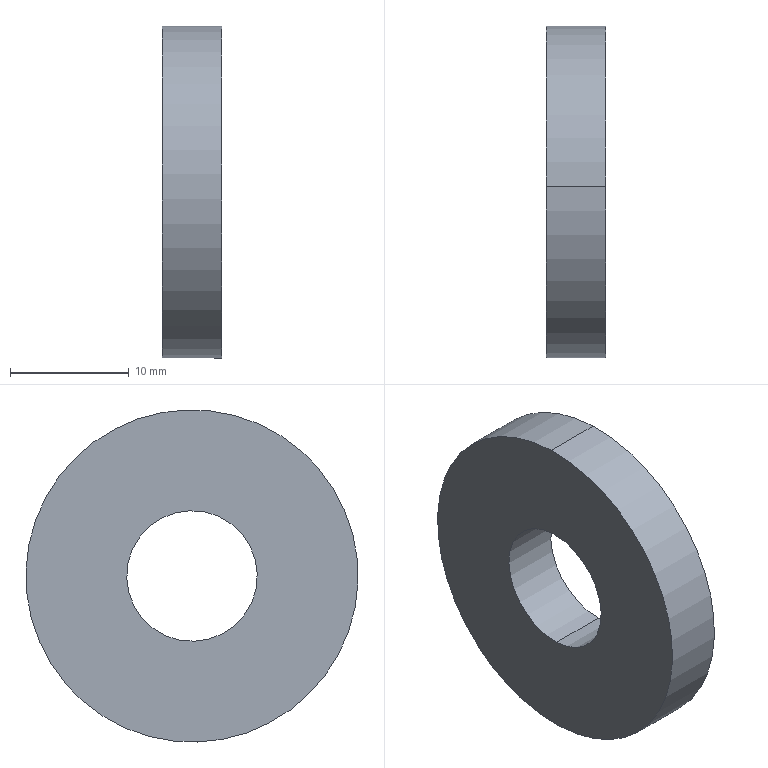Component | SolidWorks | Gasket-2 | 1 solid | 6 faces | box 5 x 28 x 28 mm | volume 2604 mm3 | cylinder 4 | plane 2 | commonest cylinder face diameters 11 x2 28 x2
build123d program:
from build123d import *

# Parameters (mm, degrees)
SKETCH1_R           = 14
SKETCH1_R_2         = 5.5
BOSS_EXTRUDE1_DEPTH = 5


with BuildPart() as part:
    # Sketch1 → Boss-Extrude1 (new body)
    with BuildSketch(Plane.XY):
        Circle(SKETCH1_R)
        Circle(SKETCH1_R_2, mode=Mode.SUBTRACT)
    extrude(amount=BOSS_EXTRUDE1_DEPTH)


solid = part.part

# Placed as in the assembly
solid = solid.moved(Location((-553.364, 0, 0), (0, 90, 0)))
STEP:
#1=CARTESIAN_POINT('',(-21.589,0.007104,0.2164));
#2=VERTEX_POINT('',#1);
#3=CARTESIAN_POINT('',(-21.589,-0.007104,-0.2164));
#4=VERTEX_POINT('',#3);
#5=CARTESIAN_POINT('',(-21.589,0.,0.));
#6=DIRECTION('',(1.,-0.,-0.));
#7=DIRECTION('',(0.,-0.03281,-0.9995));
#8=AXIS2_PLACEMENT_3D('',#5,#6,#7);
#9=CIRCLE('',#8,0.2165);
#10=EDGE_CURVE('',#2,#4,#9,.T.);
#11=ORIENTED_EDGE('',*,*,#10,.T.);
#12=CARTESIAN_POINT('',(-21.786,-0.007104,-0.2164));
#13=VERTEX_POINT('',#12);
#14=CARTESIAN_POINT('',(-21.589,-0.007104,-0.2164));
#15=DIRECTION('',(-1.,0.,0.));
#16=VECTOR('',#15,39.37);
#17=LINE('',#14,#16);
#18=EDGE_CURVE('',#4,#13,#17,.T.);
#19=ORIENTED_EDGE('',*,*,#18,.T.);
#20=CARTESIAN_POINT('',(-21.786,0.007104,0.2164));
#21=VERTEX_POINT('',#20);
#22=CARTESIAN_POINT('',(-21.786,0.,0.));
#23=DIRECTION('',(1.,-0.,-0.));
#24=DIRECTION('',(0.,-0.03281,-0.9995));
#25=AXIS2_PLACEMENT_3D('',#22,#23,#24);
#26=CIRCLE('',#25,0.2165);
#27=EDGE_CURVE('',#21,#13,#26,.T.);
#28=ORIENTED_EDGE('',*,*,#27,.F.);
#29=CARTESIAN_POINT('',(-21.589,0.007104,0.2164));
#30=DIRECTION('',(-1.,0.,0.));
#31=VECTOR('',#30,39.37);
#32=LINE('',#29,#31);
#33=EDGE_CURVE('',#2,#21,#32,.T.);
#34=ORIENTED_EDGE('',*,*,#33,.F.);
#35=EDGE_LOOP('',(#11,#19,#28,#34));
#36=FACE_OUTER_BOUND('',#35,.T.);
#37=CARTESIAN_POINT('',(-21.589,0.,0.));
#38=DIRECTION('',(-1.,0.,0.));
#39=DIRECTION('',(0.,0.03281,0.9995));
#40=AXIS2_PLACEMENT_3D('',#37,#38,#39);
#41=CYLINDRICAL_SURFACE('',#40,0.2165);
#42=ADVANCED_FACE('',(#36),#41,.F.);
#43=CARTESIAN_POINT('',(-21.589,-0.01808,-0.5509));
#44=VERTEX_POINT('',#43);
#45=CARTESIAN_POINT('',(-21.589,0.01808,0.5509));
#46=VERTEX_POINT('',#45);
#47=CARTESIAN_POINT('',(-21.589,0.,0.));
#48=DIRECTION('',(1.,-0.,-0.));
#49=DIRECTION('',(0.,-0.03281,-0.9995));
#50=AXIS2_PLACEMENT_3D('',#47,#48,#49);
#51=CIRCLE('',#50,0.5512);
#52=EDGE_CURVE('',#44,#46,#51,.T.);
#53=ORIENTED_EDGE('',*,*,#52,.F.);
#54=CARTESIAN_POINT('',(-21.786,-0.01808,-0.5509));
#55=VERTEX_POINT('',#54);
#56=CARTESIAN_POINT('',(-21.589,-0.01808,-0.5509));
#57=DIRECTION('',(-1.,0.,0.));
#58=VECTOR('',#57,39.37);
#59=LINE('',#56,#58);
#60=EDGE_CURVE('',#44,#55,#59,.T.);
#61=ORIENTED_EDGE('',*,*,#60,.T.);
#62=CARTESIAN_POINT('',(-21.786,0.01808,0.5509));
#63=VERTEX_POINT('',#62);
#64=CARTESIAN_POINT('',(-21.786,0.,0.));
#65=DIRECTION('',(1.,-0.,-0.));
#66=DIRECTION('',(0.,-0.03281,-0.9995));
#67=AXIS2_PLACEMENT_3D('',#64,#65,#66);
#68=CIRCLE('',#67,0.5512);
#69=EDGE_CURVE('',#55,#63,#68,.T.);
#70=ORIENTED_EDGE('',*,*,#69,.T.);
#71=CARTESIAN_POINT('',(-21.589,0.01808,0.5509));
#72=DIRECTION('',(-1.,0.,0.));
#73=VECTOR('',#72,39.37);
#74=LINE('',#71,#73);
#75=EDGE_CURVE('',#46,#63,#74,.T.);
#76=ORIENTED_EDGE('',*,*,#75,.F.);
#77=EDGE_LOOP('',(#53,#61,#70,#76));
#78=FACE_OUTER_BOUND('',#77,.T.);
#79=CARTESIAN_POINT('',(-21.589,0.,0.));
#80=DIRECTION('',(-1.,0.,0.));
#81=DIRECTION('',(0.,0.03281,0.9995));
#82=AXIS2_PLACEMENT_3D('',#79,#80,#81);
#83=CYLINDRICAL_SURFACE('',#82,0.5512);
#84=ADVANCED_FACE('',(#78),#83,.T.);
#85=CARTESIAN_POINT('',(-21.589,0.,0.));
#86=DIRECTION('',(1.,-0.,-0.));
#87=DIRECTION('',(0.,-0.03281,-0.9995));
#88=AXIS2_PLACEMENT_3D('',#85,#86,#87);
#89=CIRCLE('',#88,0.5512);
#90=EDGE_CURVE('',#46,#44,#89,.T.);
#91=ORIENTED_EDGE('',*,*,#90,.T.);
#92=ORIENTED_EDGE('',*,*,#52,.T.);
#93=EDGE_LOOP('',(#91,#92));
#94=FACE_OUTER_BOUND('',#93,.T.);
#95=ORIENTED_EDGE('',*,*,#10,.F.);
#96=CARTESIAN_POINT('',(-21.589,0.,0.));
#97=DIRECTION('',(1.,-0.,-0.));
#98=DIRECTION('',(0.,-0.03281,-0.9995));
#99=AXIS2_PLACEMENT_3D('',#96,#97,#98);
#100=CIRCLE('',#99,0.2165);
#101=EDGE_CURVE('',#4,#2,#100,.T.);
#102=ORIENTED_EDGE('',*,*,#101,.F.);
#103=EDGE_LOOP('',(#95,#102));
#104=FACE_BOUND('',#103,.T.);
#105=CARTESIAN_POINT('',(-21.589,0.,0.));
#106=DIRECTION('',(1.,-0.,-0.));
#107=DIRECTION('',(-0.,-0.03281,-0.9995));
#108=AXIS2_PLACEMENT_3D('',#105,#106,#107);
#109=PLANE('',#108);
#110=ADVANCED_FACE('',(#94,#104),#109,.T.);
#111=CARTESIAN_POINT('',(-21.786,0.,0.));
#112=DIRECTION('',(1.,-0.,-0.));
#113=DIRECTION('',(0.,-0.03281,-0.9995));
#114=AXIS2_PLACEMENT_3D('',#111,#112,#113);
#115=CIRCLE('',#114,0.5512);
#116=EDGE_CURVE('',#63,#55,#115,.T.);
#117=ORIENTED_EDGE('',*,*,#116,.F.);
#118=ORIENTED_EDGE('',*,*,#69,.F.);
#119=EDGE_LOOP('',(#117,#118));
#120=FACE_OUTER_BOUND('',#119,.T.);
#121=ORIENTED_EDGE('',*,*,#27,.T.);
#122=CARTESIAN_POINT('',(-21.786,0.,0.));
#123=DIRECTION('',(1.,-0.,-0.));
#124=DIRECTION('',(0.,-0.03281,-0.9995));
#125=AXIS2_PLACEMENT_3D('',#122,#123,#124);
#126=CIRCLE('',#125,0.2165);
#127=EDGE_CURVE('',#13,#21,#126,.T.);
#128=ORIENTED_EDGE('',*,*,#127,.T.);
#129=EDGE_LOOP('',(#121,#128));
#130=FACE_BOUND('',#129,.T.);
#131=CARTESIAN_POINT('',(-21.786,0.,0.));
#132=DIRECTION('',(1.,-0.,-0.));
#133=DIRECTION('',(-0.,-0.03281,-0.9995));
#134=AXIS2_PLACEMENT_3D('',#131,#132,#133);
#135=PLANE('',#134);
#136=ADVANCED_FACE('',(#120,#130),#135,.F.);
#137=ORIENTED_EDGE('',*,*,#60,.F.);
#138=ORIENTED_EDGE('',*,*,#90,.F.);
#139=ORIENTED_EDGE('',*,*,#75,.T.);
#140=ORIENTED_EDGE('',*,*,#116,.T.);
#141=EDGE_LOOP('',(#137,#138,#139,#140));
#142=FACE_OUTER_BOUND('',#141,.T.);
#143=CARTESIAN_POINT('',(-21.589,0.,0.));
#144=DIRECTION('',(-1.,0.,0.));
#145=DIRECTION('',(0.,0.03281,0.9995));
#146=AXIS2_PLACEMENT_3D('',#143,#144,#145);
#147=CYLINDRICAL_SURFACE('',#146,0.5512);
#148=ADVANCED_FACE('',(#142),#147,.T.);
#149=ORIENTED_EDGE('',*,*,#18,.F.);
#150=ORIENTED_EDGE('',*,*,#101,.T.);
#151=ORIENTED_EDGE('',*,*,#33,.T.);
#152=ORIENTED_EDGE('',*,*,#127,.F.);
#153=EDGE_LOOP('',(#149,#150,#151,#152));
#154=FACE_OUTER_BOUND('',#153,.T.);
#155=CARTESIAN_POINT('',(-21.589,0.,0.));
#156=DIRECTION('',(-1.,0.,0.));
#157=DIRECTION('',(0.,0.03281,0.9995));
#158=AXIS2_PLACEMENT_3D('',#155,#156,#157);
#159=CYLINDRICAL_SURFACE('',#158,0.2165);
#160=ADVANCED_FACE('',(#154),#159,.F.);
#161=CLOSED_SHELL('',(#42,#84,#110,#136,#148,#160));
#162=MANIFOLD_SOLID_BREP('',#161);
#163=CARTESIAN_POINT('',(0.,0.,0.));
#164=DIRECTION('',(0.,0.,1.));
#165=DIRECTION('',(1.,0.,0.));
#166=AXIS2_PLACEMENT_3D('',#163,#164,#165);
#167=(LENGTH_UNIT()NAMED_UNIT(*)SI_UNIT($,.METRE.));
#168=LENGTH_MEASURE_WITH_UNIT(LENGTH_MEASURE(0.0254),#167);
#169=DIMENSIONAL_EXPONENTS(1.,0.,0.,0.,0.,0.,0.);
#170=(CONVERSION_BASED_UNIT('',#168)LENGTH_UNIT()NAMED_UNIT(#169));
#171=UNCERTAINTY_MEASURE_WITH_UNIT(LENGTH_MEASURE(0.00001),#170,'','');
#172=(NAMED_UNIT(*)PLANE_ANGLE_UNIT()SI_UNIT($,.RADIAN.));
#173=(NAMED_UNIT(*)SI_UNIT($,.STERADIAN.)SOLID_ANGLE_UNIT());
#174=(GEOMETRIC_REPRESENTATION_CONTEXT(3)GLOBAL_UNCERTAINTY_ASSIGNED_CONTEXT((#171))GLOBAL_UNIT_ASSIGNED_CONTEXT((#170,#172,#173))REPRESENTATION_CONTEXT('',''));
#175=ADVANCED_BREP_SHAPE_REPRESENTATION('',(#162,#166),#174);
#176=COLOUR_RGB('',0.7922,0.8196,0.9333);
#177=FILL_AREA_STYLE_COLOUR('',#176);
#178=FILL_AREA_STYLE('',(#177));
#179=SURFACE_STYLE_FILL_AREA(#178);
#180=SURFACE_SIDE_STYLE('',(#179));
#181=SURFACE_STYLE_USAGE(.BOTH.,#180);
#182=PRESENTATION_STYLE_ASSIGNMENT((#181));
#183=STYLED_ITEM('',(#182),#162);
#184=PRESENTATION_LAYER_ASSIGNMENT('','',(#183));
#185=(LENGTH_UNIT()NAMED_UNIT(*)SI_UNIT($,.METRE.));
#186=LENGTH_MEASURE_WITH_UNIT(LENGTH_MEASURE(0.0254),#185);
#187=DIMENSIONAL_EXPONENTS(1.,0.,0.,0.,0.,0.,0.);
#188=(CONVERSION_BASED_UNIT('',#186)LENGTH_UNIT()NAMED_UNIT(#187));
#189=UNCERTAINTY_MEASURE_WITH_UNIT(LENGTH_MEASURE(0.00001),#188,'','');
#190=(NAMED_UNIT(*)PLANE_ANGLE_UNIT()SI_UNIT($,.RADIAN.));
#191=(NAMED_UNIT(*)SI_UNIT($,.STERADIAN.)SOLID_ANGLE_UNIT());
#192=(GEOMETRIC_REPRESENTATION_CONTEXT(3)GLOBAL_UNCERTAINTY_ASSIGNED_CONTEXT((#189))GLOBAL_UNIT_ASSIGNED_CONTEXT((#188,#190,#191))REPRESENTATION_CONTEXT('',''));
#193=MECHANICAL_DESIGN_GEOMETRIC_PRESENTATION_REPRESENTATION('',(#183),#192);